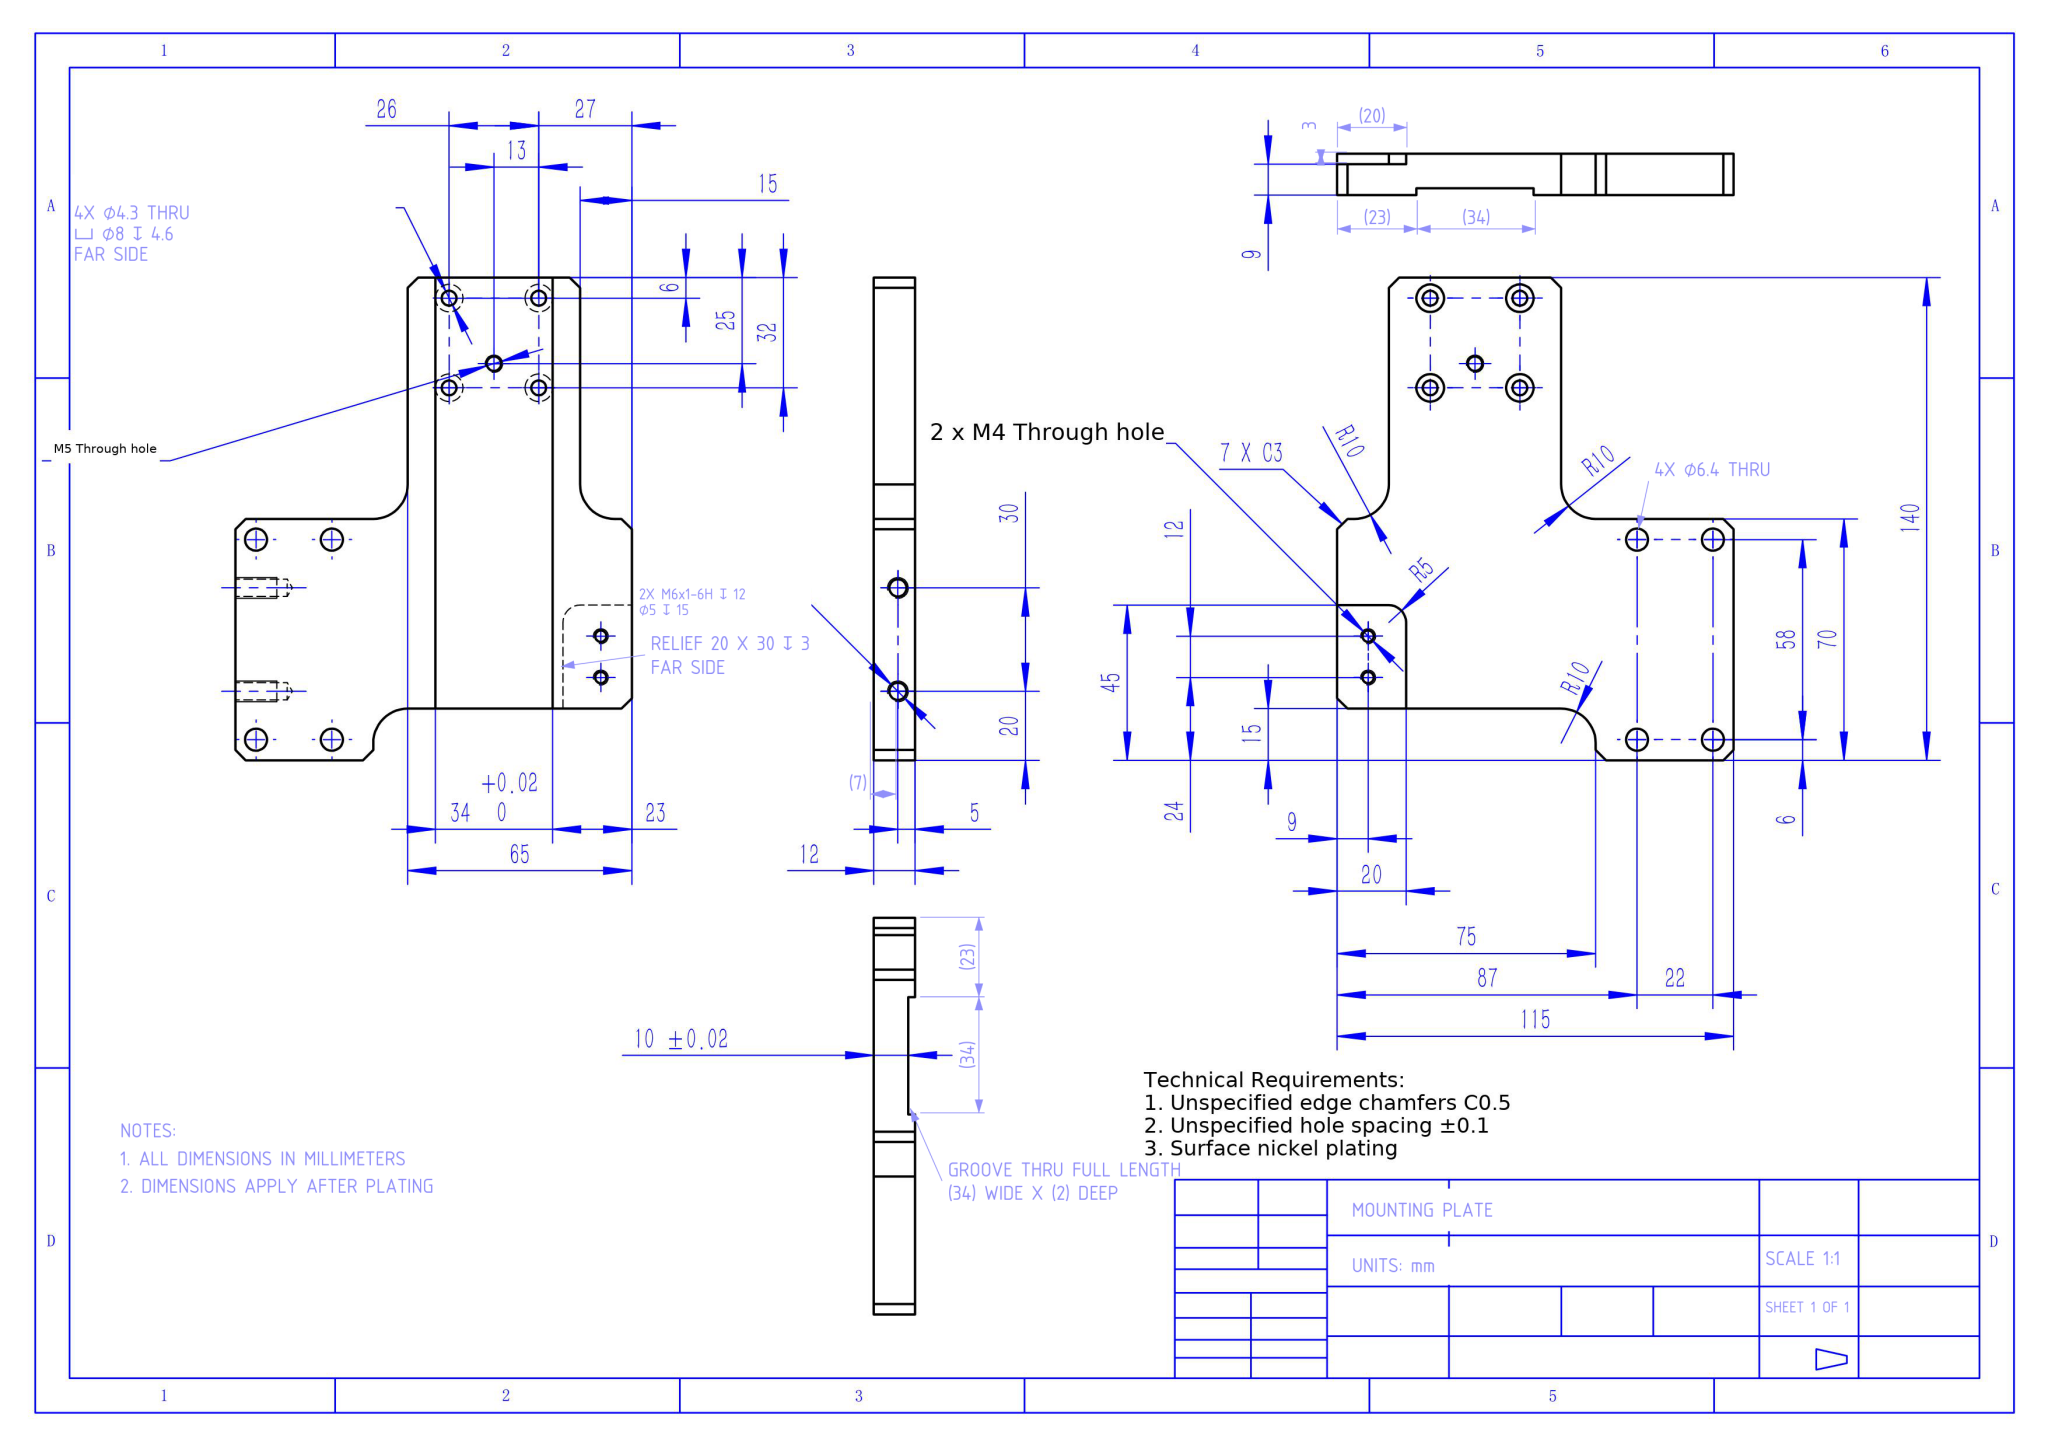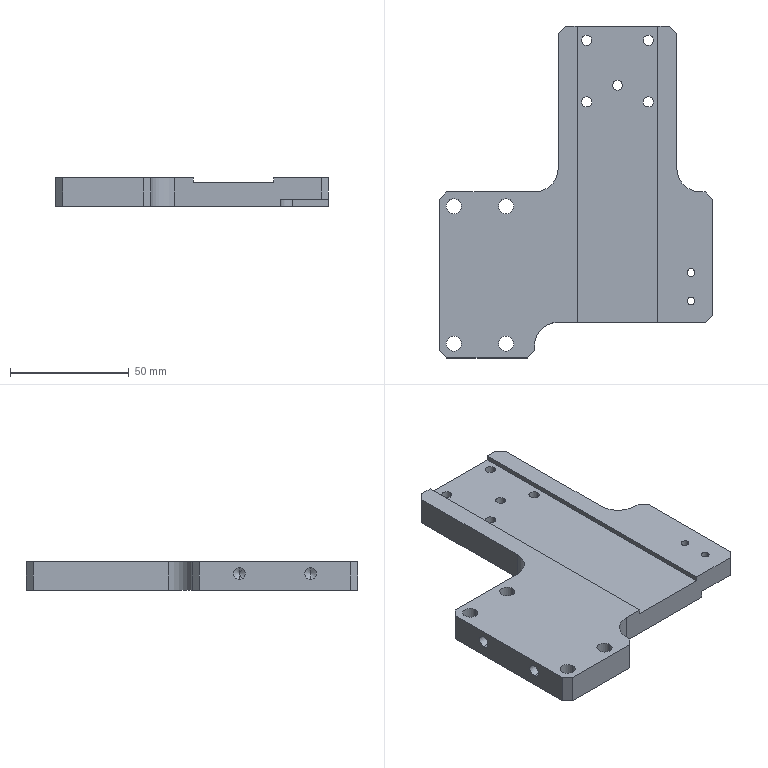Part | NX | mm | 1 solid | 72 faces | box 115 x 140 x 12 mm | volume 111540 mm3 | cylinder 38 | plane 30 | cone 4 | commonest cylinder face diameters 8 x8 4.3 x8 6.4 x8 5 x4 3.3 x4 20 x3 4.2 x2 10 x1